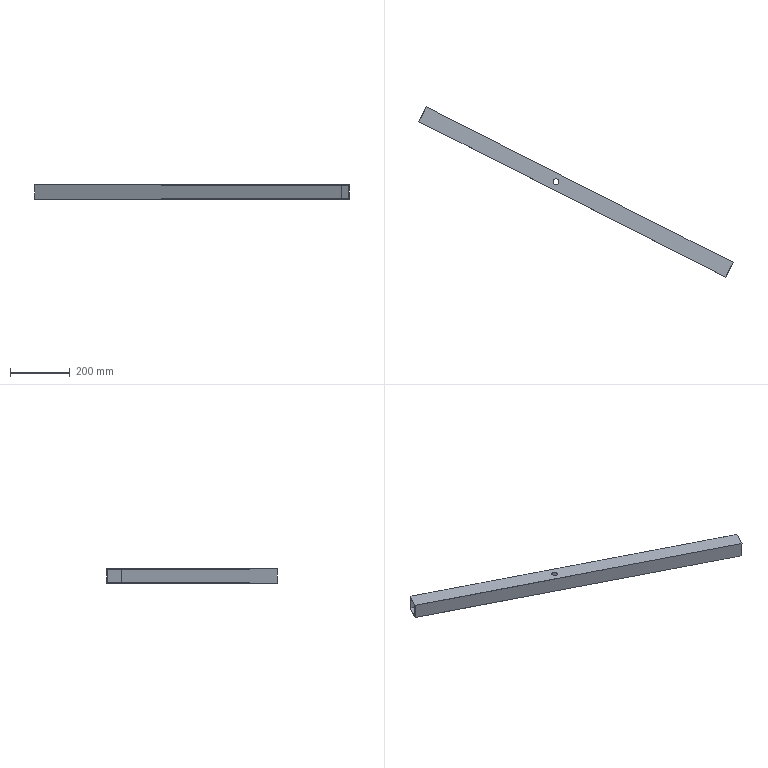Component | SolidWorks | FrameAssemblyDrawing11111-1_Part8-1 | 1 solid | 14 faces | box 1050.63 x 568.97 x 50 mm | volume 463343 mm3 | plane 10 | cylinder 4 | commonest cylinder face diameters 20 x4
build123d program:
from build123d import *

# Parameters (mm, degrees)
SKETCH2_W           = 1150
SKETCH2_H           = 55
BOSS_EXTRUDE1_DEPTH = 50
SHELL1_T            = -2
SKETCH3_R           = 10
CUT_EXTRUDE2_DEPTH  = 1091.718


with BuildPart() as part:
    # Sketch2 → Boss-Extrude1 (new body)
    with BuildSketch(Plane.XY):
        with Locations((513.859, 11.902)):
            Rectangle(SKETCH2_W, SKETCH2_H)
    extrude(amount=BOSS_EXTRUDE1_DEPTH)

    # Shell1
    shell1_openings = [part.faces().sort_by_distance(p)[0] for p in [
        (1088.859, 11.902, 25),
        (-61.141, 11.902, 25),
    ]]
    offset(amount=SHELL1_T, openings=shell1_openings, kind=Kind.INTERSECTION)

    # Sketch3 → Cut-Extrude2 (cut, through all)
    with BuildSketch(Plane.XY.offset(50)):
        with Locations((438.859, 11.902)):
            Circle(SKETCH3_R)
    extrude(amount=-CUT_EXTRUDE2_DEPTH, mode=Mode.SUBTRACT)


solid = part.part

# Placed as in the assembly
solid = solid.moved(Location((-697.013, -707.415, 1035.971), (0, 0, -26.879)))
STEP:
#1=COLOUR_RGB('',0.7922,0.8196,0.9333);
#2=FILL_AREA_STYLE_COLOUR('',#1);
#3=FILL_AREA_STYLE('',(#2));
#4=SURFACE_STYLE_FILL_AREA(#3);
#5=SURFACE_SIDE_STYLE('',(#4));
#6=SURFACE_STYLE_USAGE(.BOTH.,#5);
#7=PRESENTATION_STYLE_ASSIGNMENT((#6));
#8=CARTESIAN_POINT('',(-12.169,-35.066,42.676));
#9=VERTEX_POINT('',#8);
#10=CARTESIAN_POINT('',(-11.467,-35.422,42.676));
#11=VERTEX_POINT('',#10);
#12=CARTESIAN_POINT('',(-11.818,-35.244,42.676));
#13=DIRECTION('',(-0.,-0.,1.));
#14=DIRECTION('',(0.892,-0.4521,-0.));
#15=AXIS2_PLACEMENT_3D('',#12,#13,#14);
#16=CIRCLE('',#15,0.3937);
#17=EDGE_CURVE('',#9,#11,#16,.T.);
#18=ORIENTED_EDGE('',*,*,#17,.F.);
#19=CARTESIAN_POINT('',(-12.169,-35.066,42.755));
#20=VERTEX_POINT('',#19);
#21=CARTESIAN_POINT('',(-12.169,-35.066,40.786));
#22=DIRECTION('',(-0.,-0.,1.));
#23=VECTOR('',#22,39.37);
#24=LINE('',#21,#23);
#25=EDGE_CURVE('',#9,#20,#24,.T.);
#26=ORIENTED_EDGE('',*,*,#25,.T.);
#27=CARTESIAN_POINT('',(-11.467,-35.422,42.755));
#28=VERTEX_POINT('',#27);
#29=CARTESIAN_POINT('',(-11.818,-35.244,42.755));
#30=DIRECTION('',(-0.,-0.,1.));
#31=DIRECTION('',(0.892,-0.4521,-0.));
#32=AXIS2_PLACEMENT_3D('',#29,#30,#31);
#33=CIRCLE('',#32,0.3937);
#34=EDGE_CURVE('',#20,#28,#33,.T.);
#35=ORIENTED_EDGE('',*,*,#34,.T.);
#36=CARTESIAN_POINT('',(-11.467,-35.422,40.786));
#37=DIRECTION('',(-0.,-0.,1.));
#38=VECTOR('',#37,39.37);
#39=LINE('',#36,#38);
#40=EDGE_CURVE('',#11,#28,#39,.T.);
#41=ORIENTED_EDGE('',*,*,#40,.F.);
#42=EDGE_LOOP('',(#18,#26,#35,#41));
#43=FACE_OUTER_BOUND('',#42,.T.);
#44=CARTESIAN_POINT('',(-11.818,-35.244,40.786));
#45=DIRECTION('',(-0.,-0.,1.));
#46=DIRECTION('',(0.892,-0.4521,-0.));
#47=AXIS2_PLACEMENT_3D('',#44,#45,#46);
#48=CYLINDRICAL_SURFACE('',#47,0.3937);
#49=ADVANCED_FACE('',(#43),#48,.F.);
#50=CARTESIAN_POINT('',(-12.169,-35.066,40.786));
#51=VERTEX_POINT('',#50);
#52=CARTESIAN_POINT('',(-11.467,-35.422,40.786));
#53=VERTEX_POINT('',#52);
#54=CARTESIAN_POINT('',(-11.818,-35.244,40.786));
#55=DIRECTION('',(-0.,-0.,1.));
#56=DIRECTION('',(0.892,-0.4521,-0.));
#57=AXIS2_PLACEMENT_3D('',#54,#55,#56);
#58=CIRCLE('',#57,0.3937);
#59=EDGE_CURVE('',#51,#53,#58,.T.);
#60=ORIENTED_EDGE('',*,*,#59,.F.);
#61=CARTESIAN_POINT('',(-12.169,-35.066,40.865));
#62=VERTEX_POINT('',#61);
#63=CARTESIAN_POINT('',(-12.169,-35.066,40.786));
#64=DIRECTION('',(-0.,-0.,1.));
#65=VECTOR('',#64,39.37);
#66=LINE('',#63,#65);
#67=EDGE_CURVE('',#51,#62,#66,.T.);
#68=ORIENTED_EDGE('',*,*,#67,.T.);
#69=CARTESIAN_POINT('',(-11.467,-35.422,40.865));
#70=VERTEX_POINT('',#69);
#71=CARTESIAN_POINT('',(-11.818,-35.244,40.865));
#72=DIRECTION('',(-0.,-0.,1.));
#73=DIRECTION('',(0.892,-0.4521,-0.));
#74=AXIS2_PLACEMENT_3D('',#71,#72,#73);
#75=CIRCLE('',#74,0.3937);
#76=EDGE_CURVE('',#62,#70,#75,.T.);
#77=ORIENTED_EDGE('',*,*,#76,.T.);
#78=CARTESIAN_POINT('',(-11.467,-35.422,40.786));
#79=DIRECTION('',(-0.,-0.,1.));
#80=VECTOR('',#79,39.37);
#81=LINE('',#78,#80);
#82=EDGE_CURVE('',#53,#70,#81,.T.);
#83=ORIENTED_EDGE('',*,*,#82,.F.);
#84=EDGE_LOOP('',(#60,#68,#77,#83));
#85=FACE_OUTER_BOUND('',#84,.T.);
#86=CARTESIAN_POINT('',(-11.818,-35.244,40.786));
#87=DIRECTION('',(-0.,-0.,1.));
#88=DIRECTION('',(0.892,-0.4521,-0.));
#89=AXIS2_PLACEMENT_3D('',#86,#87,#88);
#90=CYLINDRICAL_SURFACE('',#89,0.3937);
#91=ADVANCED_FACE('',(#85),#90,.F.);
#92=CARTESIAN_POINT('',(-28.887,-25.379,40.786));
#93=VERTEX_POINT('',#92);
#94=CARTESIAN_POINT('',(-29.866,-27.31,40.786));
#95=VERTEX_POINT('',#94);
#96=CARTESIAN_POINT('',(-28.887,-25.379,40.786));
#97=DIRECTION('',(-0.4521,-0.892,-0.));
#98=VECTOR('',#97,39.37);
#99=LINE('',#96,#98);
#100=EDGE_CURVE('',#93,#95,#99,.T.);
#101=ORIENTED_EDGE('',*,*,#100,.T.);
#102=CARTESIAN_POINT('',(-29.866,-27.31,42.755));
#103=VERTEX_POINT('',#102);
#104=CARTESIAN_POINT('',(-29.866,-27.31,42.755));
#105=DIRECTION('',(0.,0.,-1.));
#106=VECTOR('',#105,39.37);
#107=LINE('',#104,#106);
#108=EDGE_CURVE('',#103,#95,#107,.T.);
#109=ORIENTED_EDGE('',*,*,#108,.F.);
#110=CARTESIAN_POINT('',(-28.887,-25.379,42.755));
#111=VERTEX_POINT('',#110);
#112=CARTESIAN_POINT('',(-28.887,-25.379,42.755));
#113=DIRECTION('',(-0.4521,-0.892,-0.));
#114=VECTOR('',#113,39.37);
#115=LINE('',#112,#114);
#116=EDGE_CURVE('',#111,#103,#115,.T.);
#117=ORIENTED_EDGE('',*,*,#116,.F.);
#118=CARTESIAN_POINT('',(-28.887,-25.379,42.755));
#119=DIRECTION('',(0.,0.,-1.));
#120=VECTOR('',#119,39.37);
#121=LINE('',#118,#120);
#122=EDGE_CURVE('',#111,#93,#121,.T.);
#123=ORIENTED_EDGE('',*,*,#122,.T.);
#124=EDGE_LOOP('',(#101,#109,#117,#123));
#125=FACE_OUTER_BOUND('',#124,.T.);
#126=CARTESIAN_POINT('',(-28.923,-25.449,40.865));
#127=VERTEX_POINT('',#126);
#128=CARTESIAN_POINT('',(-29.831,-27.24,40.865));
#129=VERTEX_POINT('',#128);
#130=CARTESIAN_POINT('',(-28.887,-25.379,40.865));
#131=DIRECTION('',(-0.4521,-0.892,-0.));
#132=VECTOR('',#131,39.37);
#133=LINE('',#130,#132);
#134=EDGE_CURVE('',#127,#129,#133,.T.);
#135=ORIENTED_EDGE('',*,*,#134,.F.);
#136=CARTESIAN_POINT('',(-28.923,-25.449,42.676));
#137=VERTEX_POINT('',#136);
#138=CARTESIAN_POINT('',(-28.923,-25.449,42.755));
#139=DIRECTION('',(0.,0.,-1.));
#140=VECTOR('',#139,39.37);
#141=LINE('',#138,#140);
#142=EDGE_CURVE('',#137,#127,#141,.T.);
#143=ORIENTED_EDGE('',*,*,#142,.F.);
#144=CARTESIAN_POINT('',(-29.831,-27.24,42.676));
#145=VERTEX_POINT('',#144);
#146=CARTESIAN_POINT('',(-28.887,-25.379,42.676));
#147=DIRECTION('',(-0.4521,-0.892,-0.));
#148=VECTOR('',#147,39.37);
#149=LINE('',#146,#148);
#150=EDGE_CURVE('',#137,#145,#149,.T.);
#151=ORIENTED_EDGE('',*,*,#150,.T.);
#152=CARTESIAN_POINT('',(-29.831,-27.24,42.755));
#153=DIRECTION('',(0.,0.,-1.));
#154=VECTOR('',#153,39.37);
#155=LINE('',#152,#154);
#156=EDGE_CURVE('',#145,#129,#155,.T.);
#157=ORIENTED_EDGE('',*,*,#156,.T.);
#158=EDGE_LOOP('',(#135,#143,#151,#157));
#159=FACE_BOUND('',#158,.T.);
#160=CARTESIAN_POINT('',(-28.887,-25.379,42.755));
#161=DIRECTION('',(0.892,-0.4521,-0.));
#162=DIRECTION('',(0.,0.,-1.));
#163=AXIS2_PLACEMENT_3D('',#160,#161,#162);
#164=PLANE('',#163);
#165=ADVANCED_FACE('',(#125,#159),#164,.F.);
#166=CARTESIAN_POINT('',(10.518,-47.78,40.786));
#167=VERTEX_POINT('',#166);
#168=CARTESIAN_POINT('',(11.497,-45.848,40.786));
#169=VERTEX_POINT('',#168);
#170=CARTESIAN_POINT('',(11.497,-45.848,40.786));
#171=DIRECTION('',(0.4521,0.892,0.));
#172=VECTOR('',#171,39.37);
#173=LINE('',#170,#172);
#174=EDGE_CURVE('',#167,#169,#173,.T.);
#175=ORIENTED_EDGE('',*,*,#174,.T.);
#176=CARTESIAN_POINT('',(11.497,-45.848,42.755));
#177=VERTEX_POINT('',#176);
#178=CARTESIAN_POINT('',(11.497,-45.848,42.755));
#179=DIRECTION('',(0.,0.,-1.));
#180=VECTOR('',#179,39.37);
#181=LINE('',#178,#180);
#182=EDGE_CURVE('',#177,#169,#181,.T.);
#183=ORIENTED_EDGE('',*,*,#182,.F.);
#184=CARTESIAN_POINT('',(10.518,-47.78,42.755));
#185=VERTEX_POINT('',#184);
#186=CARTESIAN_POINT('',(11.497,-45.848,42.755));
#187=DIRECTION('',(0.4521,0.892,0.));
#188=VECTOR('',#187,39.37);
#189=LINE('',#186,#188);
#190=EDGE_CURVE('',#185,#177,#189,.T.);
#191=ORIENTED_EDGE('',*,*,#190,.F.);
#192=CARTESIAN_POINT('',(10.518,-47.78,42.755));
#193=DIRECTION('',(0.,0.,-1.));
#194=VECTOR('',#193,39.37);
#195=LINE('',#192,#194);
#196=EDGE_CURVE('',#185,#167,#195,.T.);
#197=ORIENTED_EDGE('',*,*,#196,.T.);
#198=EDGE_LOOP('',(#175,#183,#191,#197));
#199=FACE_OUTER_BOUND('',#198,.T.);
#200=CARTESIAN_POINT('',(10.554,-47.709,40.865));
#201=VERTEX_POINT('',#200);
#202=CARTESIAN_POINT('',(11.462,-45.918,40.865));
#203=VERTEX_POINT('',#202);
#204=CARTESIAN_POINT('',(11.497,-45.848,40.865));
#205=DIRECTION('',(0.4521,0.892,0.));
#206=VECTOR('',#205,39.37);
#207=LINE('',#204,#206);
#208=EDGE_CURVE('',#201,#203,#207,.T.);
#209=ORIENTED_EDGE('',*,*,#208,.F.);
#210=CARTESIAN_POINT('',(10.554,-47.709,42.676));
#211=VERTEX_POINT('',#210);
#212=CARTESIAN_POINT('',(10.554,-47.709,42.755));
#213=DIRECTION('',(0.,0.,-1.));
#214=VECTOR('',#213,39.37);
#215=LINE('',#212,#214);
#216=EDGE_CURVE('',#211,#201,#215,.T.);
#217=ORIENTED_EDGE('',*,*,#216,.F.);
#218=CARTESIAN_POINT('',(11.462,-45.918,42.676));
#219=VERTEX_POINT('',#218);
#220=CARTESIAN_POINT('',(11.497,-45.848,42.676));
#221=DIRECTION('',(0.4521,0.892,0.));
#222=VECTOR('',#221,39.37);
#223=LINE('',#220,#222);
#224=EDGE_CURVE('',#211,#219,#223,.T.);
#225=ORIENTED_EDGE('',*,*,#224,.T.);
#226=CARTESIAN_POINT('',(11.462,-45.918,42.755));
#227=DIRECTION('',(0.,0.,-1.));
#228=VECTOR('',#227,39.37);
#229=LINE('',#226,#228);
#230=EDGE_CURVE('',#219,#203,#229,.T.);
#231=ORIENTED_EDGE('',*,*,#230,.T.);
#232=EDGE_LOOP('',(#209,#217,#225,#231));
#233=FACE_BOUND('',#232,.T.);
#234=CARTESIAN_POINT('',(11.497,-45.848,42.755));
#235=DIRECTION('',(-0.892,0.4521,0.));
#236=DIRECTION('',(-0.,-0.,1.));
#237=AXIS2_PLACEMENT_3D('',#234,#235,#236);
#238=PLANE('',#237);
#239=ADVANCED_FACE('',(#199,#233),#238,.F.);
#240=CARTESIAN_POINT('',(-29.866,-27.31,40.786));
#241=DIRECTION('',(0.892,-0.4521,-0.));
#242=VECTOR('',#241,39.37);
#243=LINE('',#240,#242);
#244=EDGE_CURVE('',#95,#167,#243,.T.);
#245=ORIENTED_EDGE('',*,*,#244,.T.);
#246=ORIENTED_EDGE('',*,*,#196,.F.);
#247=CARTESIAN_POINT('',(-29.866,-27.31,42.755));
#248=DIRECTION('',(0.892,-0.4521,-0.));
#249=VECTOR('',#248,39.37);
#250=LINE('',#247,#249);
#251=EDGE_CURVE('',#103,#185,#250,.T.);
#252=ORIENTED_EDGE('',*,*,#251,.F.);
#253=ORIENTED_EDGE('',*,*,#108,.T.);
#254=EDGE_LOOP('',(#245,#246,#252,#253));
#255=FACE_OUTER_BOUND('',#254,.T.);
#256=CARTESIAN_POINT('',(-29.866,-27.31,42.755));
#257=DIRECTION('',(0.4521,0.892,0.));
#258=DIRECTION('',(-0.,-0.,1.));
#259=AXIS2_PLACEMENT_3D('',#256,#257,#258);
#260=PLANE('',#259);
#261=ADVANCED_FACE('',(#255),#260,.F.);
#262=CARTESIAN_POINT('',(-28.887,-25.379,40.786));
#263=DIRECTION('',(-0.892,0.4521,0.));
#264=VECTOR('',#263,39.37);
#265=LINE('',#262,#264);
#266=EDGE_CURVE('',#169,#93,#265,.T.);
#267=ORIENTED_EDGE('',*,*,#266,.T.);
#268=ORIENTED_EDGE('',*,*,#122,.F.);
#269=CARTESIAN_POINT('',(-28.887,-25.379,42.755));
#270=DIRECTION('',(-0.892,0.4521,0.));
#271=VECTOR('',#270,39.37);
#272=LINE('',#269,#271);
#273=EDGE_CURVE('',#177,#111,#272,.T.);
#274=ORIENTED_EDGE('',*,*,#273,.F.);
#275=ORIENTED_EDGE('',*,*,#182,.T.);
#276=EDGE_LOOP('',(#267,#268,#274,#275));
#277=FACE_OUTER_BOUND('',#276,.T.);
#278=CARTESIAN_POINT('',(-28.887,-25.379,42.755));
#279=DIRECTION('',(-0.4521,-0.892,-0.));
#280=DIRECTION('',(0.,0.,-1.));
#281=AXIS2_PLACEMENT_3D('',#278,#279,#280);
#282=PLANE('',#281);
#283=ADVANCED_FACE('',(#277),#282,.F.);
#284=CARTESIAN_POINT('',(-11.818,-35.244,42.755));
#285=DIRECTION('',(-0.,-0.,1.));
#286=DIRECTION('',(0.892,-0.4521,-0.));
#287=AXIS2_PLACEMENT_3D('',#284,#285,#286);
#288=CIRCLE('',#287,0.3937);
#289=EDGE_CURVE('',#28,#20,#288,.T.);
#290=ORIENTED_EDGE('',*,*,#289,.F.);
#291=ORIENTED_EDGE('',*,*,#34,.F.);
#292=EDGE_LOOP('',(#290,#291));
#293=FACE_BOUND('',#292,.T.);
#294=ORIENTED_EDGE('',*,*,#116,.T.);
#295=ORIENTED_EDGE('',*,*,#251,.T.);
#296=ORIENTED_EDGE('',*,*,#190,.T.);
#297=ORIENTED_EDGE('',*,*,#273,.T.);
#298=EDGE_LOOP('',(#294,#295,#296,#297));
#299=FACE_OUTER_BOUND('',#298,.T.);
#300=CARTESIAN_POINT('',(-27.441,-27.851,42.755));
#301=DIRECTION('',(-0.,-0.,1.));
#302=DIRECTION('',(0.892,-0.4521,-0.));
#303=AXIS2_PLACEMENT_3D('',#300,#301,#302);
#304=PLANE('',#303);
#305=ADVANCED_FACE('',(#293,#299),#304,.T.);
#306=CARTESIAN_POINT('',(-11.818,-35.244,40.786));
#307=DIRECTION('',(-0.,-0.,1.));
#308=DIRECTION('',(0.892,-0.4521,-0.));
#309=AXIS2_PLACEMENT_3D('',#306,#307,#308);
#310=CIRCLE('',#309,0.3937);
#311=EDGE_CURVE('',#53,#51,#310,.T.);
#312=ORIENTED_EDGE('',*,*,#311,.T.);
#313=ORIENTED_EDGE('',*,*,#59,.T.);
#314=EDGE_LOOP('',(#312,#313));
#315=FACE_BOUND('',#314,.T.);
#316=ORIENTED_EDGE('',*,*,#100,.F.);
#317=ORIENTED_EDGE('',*,*,#266,.F.);
#318=ORIENTED_EDGE('',*,*,#174,.F.);
#319=ORIENTED_EDGE('',*,*,#244,.F.);
#320=EDGE_LOOP('',(#316,#317,#318,#319));
#321=FACE_OUTER_BOUND('',#320,.T.);
#322=CARTESIAN_POINT('',(-27.441,-27.851,40.786));
#323=DIRECTION('',(-0.,-0.,1.));
#324=DIRECTION('',(0.892,-0.4521,-0.));
#325=AXIS2_PLACEMENT_3D('',#322,#323,#324);
#326=PLANE('',#325);
#327=ADVANCED_FACE('',(#315,#321),#326,.F.);
#328=CARTESIAN_POINT('',(-29.831,-27.24,40.865));
#329=DIRECTION('',(0.892,-0.4521,-0.));
#330=VECTOR('',#329,39.37);
#331=LINE('',#328,#330);
#332=EDGE_CURVE('',#129,#201,#331,.T.);
#333=ORIENTED_EDGE('',*,*,#332,.F.);
#334=ORIENTED_EDGE('',*,*,#156,.F.);
#335=CARTESIAN_POINT('',(-29.831,-27.24,42.676));
#336=DIRECTION('',(0.892,-0.4521,-0.));
#337=VECTOR('',#336,39.37);
#338=LINE('',#335,#337);
#339=EDGE_CURVE('',#145,#211,#338,.T.);
#340=ORIENTED_EDGE('',*,*,#339,.T.);
#341=ORIENTED_EDGE('',*,*,#216,.T.);
#342=EDGE_LOOP('',(#333,#334,#340,#341));
#343=FACE_OUTER_BOUND('',#342,.T.);
#344=CARTESIAN_POINT('',(-29.831,-27.24,42.755));
#345=DIRECTION('',(0.4521,0.892,0.));
#346=DIRECTION('',(-0.,-0.,1.));
#347=AXIS2_PLACEMENT_3D('',#344,#345,#346);
#348=PLANE('',#347);
#349=ADVANCED_FACE('',(#343),#348,.T.);
#350=CARTESIAN_POINT('',(-28.923,-25.449,40.865));
#351=DIRECTION('',(-0.892,0.4521,0.));
#352=VECTOR('',#351,39.37);
#353=LINE('',#350,#352);
#354=EDGE_CURVE('',#203,#127,#353,.T.);
#355=ORIENTED_EDGE('',*,*,#354,.F.);
#356=ORIENTED_EDGE('',*,*,#230,.F.);
#357=CARTESIAN_POINT('',(-28.923,-25.449,42.676));
#358=DIRECTION('',(-0.892,0.4521,0.));
#359=VECTOR('',#358,39.37);
#360=LINE('',#357,#359);
#361=EDGE_CURVE('',#219,#137,#360,.T.);
#362=ORIENTED_EDGE('',*,*,#361,.T.);
#363=ORIENTED_EDGE('',*,*,#142,.T.);
#364=EDGE_LOOP('',(#355,#356,#362,#363));
#365=FACE_OUTER_BOUND('',#364,.T.);
#366=CARTESIAN_POINT('',(-28.923,-25.449,42.755));
#367=DIRECTION('',(-0.4521,-0.892,-0.));
#368=DIRECTION('',(0.,0.,-1.));
#369=AXIS2_PLACEMENT_3D('',#366,#367,#368);
#370=PLANE('',#369);
#371=ADVANCED_FACE('',(#365),#370,.T.);
#372=CARTESIAN_POINT('',(-11.818,-35.244,42.676));
#373=DIRECTION('',(-0.,-0.,1.));
#374=DIRECTION('',(0.892,-0.4521,-0.));
#375=AXIS2_PLACEMENT_3D('',#372,#373,#374);
#376=CIRCLE('',#375,0.3937);
#377=EDGE_CURVE('',#11,#9,#376,.T.);
#378=ORIENTED_EDGE('',*,*,#377,.T.);
#379=ORIENTED_EDGE('',*,*,#17,.T.);
#380=EDGE_LOOP('',(#378,#379));
#381=FACE_BOUND('',#380,.T.);
#382=ORIENTED_EDGE('',*,*,#150,.F.);
#383=ORIENTED_EDGE('',*,*,#361,.F.);
#384=ORIENTED_EDGE('',*,*,#224,.F.);
#385=ORIENTED_EDGE('',*,*,#339,.F.);
#386=EDGE_LOOP('',(#382,#383,#384,#385));
#387=FACE_OUTER_BOUND('',#386,.T.);
#388=CARTESIAN_POINT('',(-27.441,-27.851,42.676));
#389=DIRECTION('',(-0.,-0.,1.));
#390=DIRECTION('',(0.892,-0.4521,-0.));
#391=AXIS2_PLACEMENT_3D('',#388,#389,#390);
#392=PLANE('',#391);
#393=ADVANCED_FACE('',(#381,#387),#392,.F.);
#394=CARTESIAN_POINT('',(-11.818,-35.244,40.865));
#395=DIRECTION('',(-0.,-0.,1.));
#396=DIRECTION('',(0.892,-0.4521,-0.));
#397=AXIS2_PLACEMENT_3D('',#394,#395,#396);
#398=CIRCLE('',#397,0.3937);
#399=EDGE_CURVE('',#70,#62,#398,.T.);
#400=ORIENTED_EDGE('',*,*,#399,.F.);
#401=ORIENTED_EDGE('',*,*,#76,.F.);
#402=EDGE_LOOP('',(#400,#401));
#403=FACE_BOUND('',#402,.T.);
#404=ORIENTED_EDGE('',*,*,#134,.T.);
#405=ORIENTED_EDGE('',*,*,#332,.T.);
#406=ORIENTED_EDGE('',*,*,#208,.T.);
#407=ORIENTED_EDGE('',*,*,#354,.T.);
#408=EDGE_LOOP('',(#404,#405,#406,#407));
#409=FACE_OUTER_BOUND('',#408,.T.);
#410=CARTESIAN_POINT('',(-27.441,-27.851,40.865));
#411=DIRECTION('',(-0.,-0.,1.));
#412=DIRECTION('',(0.892,-0.4521,-0.));
#413=AXIS2_PLACEMENT_3D('',#410,#411,#412);
#414=PLANE('',#413);
#415=ADVANCED_FACE('',(#403,#409),#414,.T.);
#416=ORIENTED_EDGE('',*,*,#67,.F.);
#417=ORIENTED_EDGE('',*,*,#311,.F.);
#418=ORIENTED_EDGE('',*,*,#82,.T.);
#419=ORIENTED_EDGE('',*,*,#399,.T.);
#420=EDGE_LOOP('',(#416,#417,#418,#419));
#421=FACE_OUTER_BOUND('',#420,.T.);
#422=CARTESIAN_POINT('',(-11.818,-35.244,40.786));
#423=DIRECTION('',(-0.,-0.,1.));
#424=DIRECTION('',(0.892,-0.4521,-0.));
#425=AXIS2_PLACEMENT_3D('',#422,#423,#424);
#426=CYLINDRICAL_SURFACE('',#425,0.3937);
#427=ADVANCED_FACE('',(#421),#426,.F.);
#428=ORIENTED_EDGE('',*,*,#25,.F.);
#429=ORIENTED_EDGE('',*,*,#377,.F.);
#430=ORIENTED_EDGE('',*,*,#40,.T.);
#431=ORIENTED_EDGE('',*,*,#289,.T.);
#432=EDGE_LOOP('',(#428,#429,#430,#431));
#433=FACE_OUTER_BOUND('',#432,.T.);
#434=CARTESIAN_POINT('',(-11.818,-35.244,40.786));
#435=DIRECTION('',(-0.,-0.,1.));
#436=DIRECTION('',(0.892,-0.4521,-0.));
#437=AXIS2_PLACEMENT_3D('',#434,#435,#436);
#438=CYLINDRICAL_SURFACE('',#437,0.3937);
#439=ADVANCED_FACE('',(#433),#438,.F.);
#440=CLOSED_SHELL('',(#49,#91,#165,#239,#261,#283,#305,#327,#349,#371,#393,#415,#427,#439));
#441=MANIFOLD_SOLID_BREP('',#440);
#442=STYLED_ITEM('',(#7),#441);
#443=PRESENTATION_LAYER_ASSIGNMENT('','',(#442));
#444=CARTESIAN_POINT('',(0.,0.,0.));
#445=DIRECTION('',(0.,0.,1.));
#446=DIRECTION('',(1.,0.,0.));
#447=AXIS2_PLACEMENT_3D('',#444,#445,#446);
#448=(LENGTH_UNIT()NAMED_UNIT(*)SI_UNIT($,.METRE.));
#449=LENGTH_MEASURE_WITH_UNIT(LENGTH_MEASURE(0.0254),#448);
#450=DIMENSIONAL_EXPONENTS(1.,0.,0.,0.,0.,0.,0.);
#451=(CONVERSION_BASED_UNIT('',#449)LENGTH_UNIT()NAMED_UNIT(#450));
#452=UNCERTAINTY_MEASURE_WITH_UNIT(LENGTH_MEASURE(0.00001),#451,'','');
#453=(NAMED_UNIT(*)PLANE_ANGLE_UNIT()SI_UNIT($,.RADIAN.));
#454=(NAMED_UNIT(*)SI_UNIT($,.STERADIAN.)SOLID_ANGLE_UNIT());
#455=(GEOMETRIC_REPRESENTATION_CONTEXT(3)GLOBAL_UNCERTAINTY_ASSIGNED_CONTEXT((#452))GLOBAL_UNIT_ASSIGNED_CONTEXT((#451,#453,#454))REPRESENTATION_CONTEXT('',''));
#456=ADVANCED_BREP_SHAPE_REPRESENTATION('',(#441,#447),#455);
#457=(LENGTH_UNIT()NAMED_UNIT(*)SI_UNIT($,.METRE.));
#458=LENGTH_MEASURE_WITH_UNIT(LENGTH_MEASURE(0.0254),#457);
#459=DIMENSIONAL_EXPONENTS(1.,0.,0.,0.,0.,0.,0.);
#460=(CONVERSION_BASED_UNIT('',#458)LENGTH_UNIT()NAMED_UNIT(#459));
#461=UNCERTAINTY_MEASURE_WITH_UNIT(LENGTH_MEASURE(0.00001),#460,'','');
#462=(NAMED_UNIT(*)PLANE_ANGLE_UNIT()SI_UNIT($,.RADIAN.));
#463=(NAMED_UNIT(*)SI_UNIT($,.STERADIAN.)SOLID_ANGLE_UNIT());
#464=(GEOMETRIC_REPRESENTATION_CONTEXT(3)GLOBAL_UNCERTAINTY_ASSIGNED_CONTEXT((#461))GLOBAL_UNIT_ASSIGNED_CONTEXT((#460,#462,#463))REPRESENTATION_CONTEXT('',''));
#465=MECHANICAL_DESIGN_GEOMETRIC_PRESENTATION_REPRESENTATION('',(#442),#464);